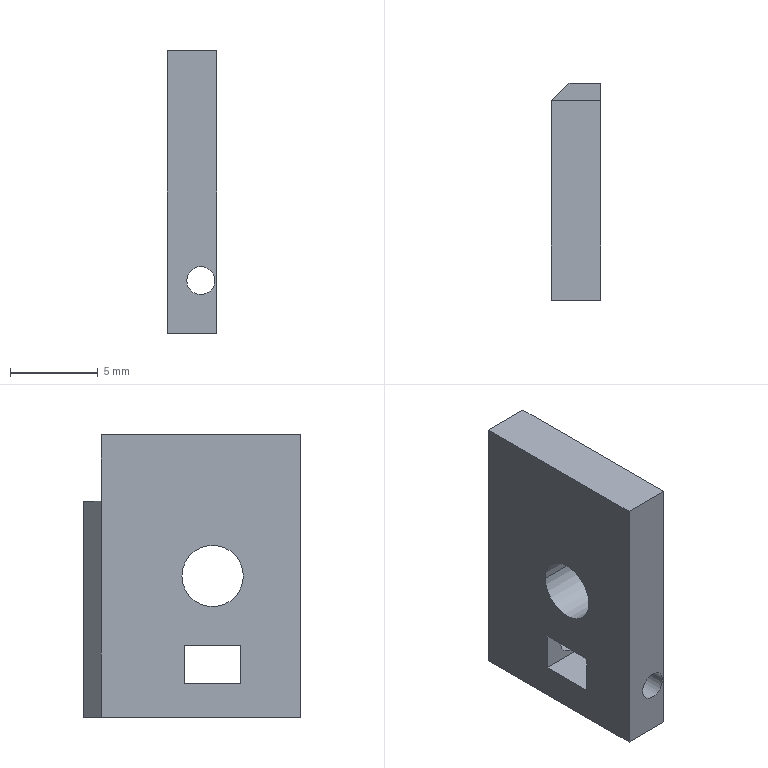Component | SolidWorks | 7.1.02.0001.00.00-0083-1 | 1 solid | 19 faces | box 2.8 x 12.35 x 16.1 mm | volume 475 mm3 | plane 13 | cylinder 6 | commonest cylinder face diameters 1.6 x4 3.5 x2
build123d program:
from build123d import *

# Parameters (mm, degrees)
SKETCH1_W           = 12.35
SKETCH1_H           = 16.1
SKETCH1_R           = 1.75
BOSS_EXTRUDE1_DEPTH = 2.8
SKETCH2_W           = 1
SKETCH2_H           = 3.8
CUT_EXTRUDE1_DEPTH  = 11.525
CHAMFER1_SIZE       = 1
SKETCH3_R           = 0.8
CUT_EXTRUDE2_DEPTH  = 16.005
SKETCH4_W           = 3.2
SKETCH4_H           = 2.2
CUT_EXTRUDE3_DEPTH  = 11.525


with BuildPart() as part:
    # Sketch1 → Boss-Extrude1 (new body)
    with BuildSketch(Plane.XY):
        Rectangle(SKETCH1_W, SKETCH1_H)
        with Locations((-1.175, 0)):
            Circle(SKETCH1_R, mode=Mode.SUBTRACT)
    extrude(amount=BOSS_EXTRUDE1_DEPTH)

    # Sketch2 → Cut-Extrude1 (cut, through all)
    with BuildSketch(Plane(origin=(0, 0, 0), x_dir=(-1, 0, 0), z_dir=(0, 0, -1))):
        with Locations((-5.675, 6.15)):
            Rectangle(SKETCH2_W, SKETCH2_H)
    extrude(amount=-CUT_EXTRUDE1_DEPTH, mode=Mode.SUBTRACT)

    # Chamfer1
    chamfer1_edges = [part.edges().sort_by_distance(p)[0] for p in [
        (6.175, -1.9, 0),
    ]]
    chamfer(chamfer1_edges, length=CHAMFER1_SIZE)

    # Sketch3 → Cut-Extrude2 (cut, through all)
    with BuildSketch(Plane.ZY.offset(6.175)):
        with Locations((1.9, -5.05)):
            Circle(SKETCH3_R)
    extrude(amount=-CUT_EXTRUDE2_DEPTH, mode=Mode.SUBTRACT)

    # Sketch4 → Cut-Extrude3 (cut, through all)
    with BuildSketch(Plane(origin=(0, 0, 0), x_dir=(-1, 0, 0), z_dir=(0, 0, -1))):
        with Locations((1.175, -5.05)):
            Rectangle(SKETCH4_W, SKETCH4_H)
    extrude(amount=-CUT_EXTRUDE3_DEPTH, mode=Mode.SUBTRACT)


solid = part.part

# Placed as in the assembly
solid = solid.moved(Location((-67.964, 9.491, 0), (90, 90, 0)))
STEP:
#1=COLOUR_RGB('',0.7922,0.8196,0.9333);
#2=FILL_AREA_STYLE_COLOUR('',#1);
#3=FILL_AREA_STYLE('',(#2));
#4=SURFACE_STYLE_FILL_AREA(#3);
#5=SURFACE_SIDE_STYLE('',(#4));
#6=SURFACE_STYLE_USAGE(.BOTH.,#5);
#7=PRESENTATION_STYLE_ASSIGNMENT((#6));
#8=CARTESIAN_POINT('',(-2.569,0.2644,-0.1988));
#9=VERTEX_POINT('',#8);
#10=CARTESIAN_POINT('',(-2.632,0.2644,-0.1988));
#11=VERTEX_POINT('',#10);
#12=CARTESIAN_POINT('',(-2.601,0.2644,-0.1988));
#13=DIRECTION('',(0.,1.,-0.));
#14=DIRECTION('',(0.,0.,-1.));
#15=AXIS2_PLACEMENT_3D('',#12,#13,#14);
#16=CIRCLE('',#15,0.0315);
#17=EDGE_CURVE('',#9,#11,#16,.T.);
#18=ORIENTED_EDGE('',*,*,#17,.T.);
#19=CARTESIAN_POINT('',(-2.632,0.1306,-0.1988));
#20=VERTEX_POINT('',#19);
#21=CARTESIAN_POINT('',(-2.632,0.6168,-0.1988));
#22=DIRECTION('',(-0.,-1.,-0.));
#23=VECTOR('',#22,39.37);
#24=LINE('',#21,#23);
#25=EDGE_CURVE('',#11,#20,#24,.T.);
#26=ORIENTED_EDGE('',*,*,#25,.T.);
#27=CARTESIAN_POINT('',(-2.569,0.1306,-0.1988));
#28=VERTEX_POINT('',#27);
#29=CARTESIAN_POINT('',(-2.601,0.1306,-0.1988));
#30=DIRECTION('',(-0.,-1.,-0.));
#31=DIRECTION('',(1.,0.,0.));
#32=AXIS2_PLACEMENT_3D('',#29,#30,#31);
#33=CIRCLE('',#32,0.0315);
#34=EDGE_CURVE('',#20,#28,#33,.T.);
#35=ORIENTED_EDGE('',*,*,#34,.T.);
#36=CARTESIAN_POINT('',(-2.569,0.6168,-0.1988));
#37=DIRECTION('',(-0.,-1.,-0.));
#38=VECTOR('',#37,39.37);
#39=LINE('',#36,#38);
#40=EDGE_CURVE('',#9,#28,#39,.T.);
#41=ORIENTED_EDGE('',*,*,#40,.F.);
#42=EDGE_LOOP('',(#18,#26,#35,#41));
#43=FACE_OUTER_BOUND('',#42,.T.);
#44=CARTESIAN_POINT('',(-2.601,0.6168,-0.1988));
#45=DIRECTION('',(-0.,-1.,-0.));
#46=DIRECTION('',(1.,0.,0.));
#47=AXIS2_PLACEMENT_3D('',#44,#45,#46);
#48=CYLINDRICAL_SURFACE('',#47,0.0315);
#49=ADVANCED_FACE('',(#43),#48,.F.);
#50=CARTESIAN_POINT('',(-2.566,0.2585,-0.));
#51=VERTEX_POINT('',#50);
#52=CARTESIAN_POINT('',(-2.566,0.3963,-0.));
#53=VERTEX_POINT('',#52);
#54=CARTESIAN_POINT('',(-2.566,0.3274,-0.));
#55=DIRECTION('',(1.,-0.,-0.));
#56=DIRECTION('',(0.,1.,0.));
#57=AXIS2_PLACEMENT_3D('',#54,#55,#56);
#58=CIRCLE('',#57,0.0689);
#59=EDGE_CURVE('',#51,#53,#58,.T.);
#60=ORIENTED_EDGE('',*,*,#59,.T.);
#61=CARTESIAN_POINT('',(-2.676,0.3963,-0.));
#62=VERTEX_POINT('',#61);
#63=CARTESIAN_POINT('',(-2.566,0.3963,-0.));
#64=DIRECTION('',(-1.,0.,0.));
#65=VECTOR('',#64,39.37);
#66=LINE('',#63,#65);
#67=EDGE_CURVE('',#53,#62,#66,.T.);
#68=ORIENTED_EDGE('',*,*,#67,.T.);
#69=CARTESIAN_POINT('',(-2.676,0.2585,-0.));
#70=VERTEX_POINT('',#69);
#71=CARTESIAN_POINT('',(-2.676,0.3274,-0.));
#72=DIRECTION('',(1.,-0.,-0.));
#73=DIRECTION('',(0.,1.,0.));
#74=AXIS2_PLACEMENT_3D('',#71,#72,#73);
#75=CIRCLE('',#74,0.0689);
#76=EDGE_CURVE('',#70,#62,#75,.T.);
#77=ORIENTED_EDGE('',*,*,#76,.F.);
#78=CARTESIAN_POINT('',(-2.566,0.2585,-0.));
#79=DIRECTION('',(-1.,0.,0.));
#80=VECTOR('',#79,39.37);
#81=LINE('',#78,#80);
#82=EDGE_CURVE('',#51,#70,#81,.T.);
#83=ORIENTED_EDGE('',*,*,#82,.F.);
#84=EDGE_LOOP('',(#60,#68,#77,#83));
#85=FACE_OUTER_BOUND('',#84,.T.);
#86=CARTESIAN_POINT('',(-2.566,0.3274,-0.));
#87=DIRECTION('',(-1.,0.,0.));
#88=DIRECTION('',(0.,-1.,-0.));
#89=AXIS2_PLACEMENT_3D('',#86,#87,#88);
#90=CYLINDRICAL_SURFACE('',#89,0.0689);
#91=ADVANCED_FACE('',(#85),#90,.F.);
#92=CARTESIAN_POINT('',(-2.632,0.6168,-0.1988));
#93=VERTEX_POINT('',#92);
#94=CARTESIAN_POINT('',(-2.569,0.6168,-0.1988));
#95=VERTEX_POINT('',#94);
#96=CARTESIAN_POINT('',(-2.601,0.6168,-0.1988));
#97=DIRECTION('',(-0.,-1.,-0.));
#98=DIRECTION('',(1.,0.,0.));
#99=AXIS2_PLACEMENT_3D('',#96,#97,#98);
#100=CIRCLE('',#99,0.0315);
#101=EDGE_CURVE('',#93,#95,#100,.T.);
#102=ORIENTED_EDGE('',*,*,#101,.F.);
#103=CARTESIAN_POINT('',(-2.632,0.3904,-0.1988));
#104=VERTEX_POINT('',#103);
#105=CARTESIAN_POINT('',(-2.632,0.6168,-0.1988));
#106=DIRECTION('',(-0.,-1.,-0.));
#107=VECTOR('',#106,39.37);
#108=LINE('',#105,#107);
#109=EDGE_CURVE('',#93,#104,#108,.T.);
#110=ORIENTED_EDGE('',*,*,#109,.T.);
#111=CARTESIAN_POINT('',(-2.569,0.3904,-0.1988));
#112=VERTEX_POINT('',#111);
#113=CARTESIAN_POINT('',(-2.601,0.3904,-0.1988));
#114=DIRECTION('',(-0.,-1.,-0.));
#115=DIRECTION('',(-1.,0.,0.));
#116=AXIS2_PLACEMENT_3D('',#113,#114,#115);
#117=CIRCLE('',#116,0.0315);
#118=EDGE_CURVE('',#104,#112,#117,.T.);
#119=ORIENTED_EDGE('',*,*,#118,.T.);
#120=CARTESIAN_POINT('',(-2.569,0.6168,-0.1988));
#121=DIRECTION('',(-0.,-1.,-0.));
#122=VECTOR('',#121,39.37);
#123=LINE('',#120,#122);
#124=EDGE_CURVE('',#95,#112,#123,.T.);
#125=ORIENTED_EDGE('',*,*,#124,.F.);
#126=EDGE_LOOP('',(#102,#110,#119,#125));
#127=FACE_OUTER_BOUND('',#126,.T.);
#128=CARTESIAN_POINT('',(-2.601,0.6168,-0.1988));
#129=DIRECTION('',(-0.,-1.,-0.));
#130=DIRECTION('',(1.,0.,0.));
#131=AXIS2_PLACEMENT_3D('',#128,#129,#130);
#132=CYLINDRICAL_SURFACE('',#131,0.0315);
#133=ADVANCED_FACE('',(#127),#132,.F.);
#134=ORIENTED_EDGE('',*,*,#109,.F.);
#135=CARTESIAN_POINT('',(-2.601,0.6168,-0.1988));
#136=DIRECTION('',(-0.,-1.,-0.));
#137=DIRECTION('',(1.,0.,0.));
#138=AXIS2_PLACEMENT_3D('',#135,#136,#137);
#139=CIRCLE('',#138,0.0315);
#140=EDGE_CURVE('',#95,#93,#139,.T.);
#141=ORIENTED_EDGE('',*,*,#140,.F.);
#142=ORIENTED_EDGE('',*,*,#124,.T.);
#143=CARTESIAN_POINT('',(-2.601,0.3904,-0.1988));
#144=DIRECTION('',(-0.,-1.,-0.));
#145=DIRECTION('',(-1.,0.,0.));
#146=AXIS2_PLACEMENT_3D('',#143,#144,#145);
#147=CIRCLE('',#146,0.0315);
#148=EDGE_CURVE('',#112,#104,#147,.T.);
#149=ORIENTED_EDGE('',*,*,#148,.T.);
#150=EDGE_LOOP('',(#134,#141,#142,#149));
#151=FACE_OUTER_BOUND('',#150,.T.);
#152=CARTESIAN_POINT('',(-2.601,0.6168,-0.1988));
#153=DIRECTION('',(-0.,-1.,-0.));
#154=DIRECTION('',(1.,0.,0.));
#155=AXIS2_PLACEMENT_3D('',#152,#153,#154);
#156=CYLINDRICAL_SURFACE('',#155,0.0315);
#157=ADVANCED_FACE('',(#151),#156,.F.);
#158=CARTESIAN_POINT('',(-2.566,0.3904,-0.1555));
#159=VERTEX_POINT('',#158);
#160=CARTESIAN_POINT('',(-2.566,0.3904,-0.2421));
#161=VERTEX_POINT('',#160);
#162=CARTESIAN_POINT('',(-2.566,0.3904,-0.1555));
#163=DIRECTION('',(-0.,0.,-1.));
#164=VECTOR('',#163,39.37);
#165=LINE('',#162,#164);
#166=EDGE_CURVE('',#159,#161,#165,.T.);
#167=ORIENTED_EDGE('',*,*,#166,.T.);
#168=CARTESIAN_POINT('',(-2.566,0.2644,-0.2421));
#169=VERTEX_POINT('',#168);
#170=CARTESIAN_POINT('',(-2.566,0.3904,-0.2421));
#171=DIRECTION('',(-0.,-1.,-0.));
#172=VECTOR('',#171,39.37);
#173=LINE('',#170,#172);
#174=EDGE_CURVE('',#161,#169,#173,.T.);
#175=ORIENTED_EDGE('',*,*,#174,.T.);
#176=CARTESIAN_POINT('',(-2.566,0.2644,-0.1555));
#177=VERTEX_POINT('',#176);
#178=CARTESIAN_POINT('',(-2.566,0.2644,-0.1555));
#179=DIRECTION('',(0.,0.,1.));
#180=VECTOR('',#179,39.37);
#181=LINE('',#178,#180);
#182=EDGE_CURVE('',#169,#177,#181,.T.);
#183=ORIENTED_EDGE('',*,*,#182,.T.);
#184=CARTESIAN_POINT('',(-2.566,0.3904,-0.1555));
#185=DIRECTION('',(0.,1.,0.));
#186=VECTOR('',#185,39.37);
#187=LINE('',#184,#186);
#188=EDGE_CURVE('',#177,#159,#187,.T.);
#189=ORIENTED_EDGE('',*,*,#188,.T.);
#190=EDGE_LOOP('',(#167,#175,#183,#189));
#191=FACE_BOUND('',#190,.T.);
#192=CARTESIAN_POINT('',(-2.566,0.5774,0.1673));
#193=VERTEX_POINT('',#192);
#194=CARTESIAN_POINT('',(-2.566,0.5774,0.3169));
#195=VERTEX_POINT('',#194);
#196=CARTESIAN_POINT('',(-2.566,0.5774,0.1673));
#197=DIRECTION('',(0.,-0.,1.));
#198=VECTOR('',#197,39.37);
#199=LINE('',#196,#198);
#200=EDGE_CURVE('',#193,#195,#199,.T.);
#201=ORIENTED_EDGE('',*,*,#200,.T.);
#202=CARTESIAN_POINT('',(-2.566,0.1306,0.3169));
#203=VERTEX_POINT('',#202);
#204=CARTESIAN_POINT('',(-2.566,0.1306,0.3169));
#205=DIRECTION('',(-0.,-1.,-0.));
#206=VECTOR('',#205,39.37);
#207=LINE('',#204,#206);
#208=EDGE_CURVE('',#195,#203,#207,.T.);
#209=ORIENTED_EDGE('',*,*,#208,.T.);
#210=CARTESIAN_POINT('',(-2.566,0.1306,-0.3169));
#211=VERTEX_POINT('',#210);
#212=CARTESIAN_POINT('',(-2.566,0.1306,0.3169));
#213=DIRECTION('',(-0.,0.,-1.));
#214=VECTOR('',#213,39.37);
#215=LINE('',#212,#214);
#216=EDGE_CURVE('',#203,#211,#215,.T.);
#217=ORIENTED_EDGE('',*,*,#216,.T.);
#218=CARTESIAN_POINT('',(-2.566,0.6168,-0.3169));
#219=VERTEX_POINT('',#218);
#220=CARTESIAN_POINT('',(-2.566,0.1306,-0.3169));
#221=DIRECTION('',(0.,1.,0.));
#222=VECTOR('',#221,39.37);
#223=LINE('',#220,#222);
#224=EDGE_CURVE('',#211,#219,#223,.T.);
#225=ORIENTED_EDGE('',*,*,#224,.T.);
#226=CARTESIAN_POINT('',(-2.566,0.6168,0.1673));
#227=VERTEX_POINT('',#226);
#228=CARTESIAN_POINT('',(-2.566,0.6168,0.3169));
#229=DIRECTION('',(0.,-0.,1.));
#230=VECTOR('',#229,39.37);
#231=LINE('',#228,#230);
#232=EDGE_CURVE('',#219,#227,#231,.T.);
#233=ORIENTED_EDGE('',*,*,#232,.T.);
#234=CARTESIAN_POINT('',(-2.566,0.6168,0.1673));
#235=DIRECTION('',(-0.,-1.,-0.));
#236=VECTOR('',#235,39.37);
#237=LINE('',#234,#236);
#238=EDGE_CURVE('',#227,#193,#237,.T.);
#239=ORIENTED_EDGE('',*,*,#238,.T.);
#240=EDGE_LOOP('',(#201,#209,#217,#225,#233,#239));
#241=FACE_OUTER_BOUND('',#240,.T.);
#242=ORIENTED_EDGE('',*,*,#59,.F.);
#243=CARTESIAN_POINT('',(-2.566,0.3274,-0.));
#244=DIRECTION('',(1.,-0.,-0.));
#245=DIRECTION('',(0.,1.,0.));
#246=AXIS2_PLACEMENT_3D('',#243,#244,#245);
#247=CIRCLE('',#246,0.0689);
#248=EDGE_CURVE('',#53,#51,#247,.T.);
#249=ORIENTED_EDGE('',*,*,#248,.F.);
#250=EDGE_LOOP('',(#242,#249));
#251=FACE_BOUND('',#250,.T.);
#252=CARTESIAN_POINT('',(-2.566,0.3737,-0.));
#253=DIRECTION('',(1.,-0.,-0.));
#254=DIRECTION('',(0.,1.,0.));
#255=AXIS2_PLACEMENT_3D('',#252,#253,#254);
#256=PLANE('',#255);
#257=ADVANCED_FACE('',(#191,#241,#251),#256,.T.);
#258=CARTESIAN_POINT('',(-2.676,0.3904,-0.2421));
#259=VERTEX_POINT('',#258);
#260=CARTESIAN_POINT('',(-2.676,0.2644,-0.2421));
#261=VERTEX_POINT('',#260);
#262=CARTESIAN_POINT('',(-2.676,0.3904,-0.2421));
#263=DIRECTION('',(-0.,-1.,-0.));
#264=VECTOR('',#263,39.37);
#265=LINE('',#262,#264);
#266=EDGE_CURVE('',#259,#261,#265,.T.);
#267=ORIENTED_EDGE('',*,*,#266,.F.);
#268=CARTESIAN_POINT('',(-2.676,0.3904,-0.1555));
#269=VERTEX_POINT('',#268);
#270=CARTESIAN_POINT('',(-2.676,0.3904,-0.1555));
#271=DIRECTION('',(-0.,0.,-1.));
#272=VECTOR('',#271,39.37);
#273=LINE('',#270,#272);
#274=EDGE_CURVE('',#269,#259,#273,.T.);
#275=ORIENTED_EDGE('',*,*,#274,.F.);
#276=CARTESIAN_POINT('',(-2.676,0.2644,-0.1555));
#277=VERTEX_POINT('',#276);
#278=CARTESIAN_POINT('',(-2.676,0.3904,-0.1555));
#279=DIRECTION('',(0.,1.,0.));
#280=VECTOR('',#279,39.37);
#281=LINE('',#278,#280);
#282=EDGE_CURVE('',#277,#269,#281,.T.);
#283=ORIENTED_EDGE('',*,*,#282,.F.);
#284=CARTESIAN_POINT('',(-2.676,0.2644,-0.1555));
#285=DIRECTION('',(0.,0.,1.));
#286=VECTOR('',#285,39.37);
#287=LINE('',#284,#286);
#288=EDGE_CURVE('',#261,#277,#287,.T.);
#289=ORIENTED_EDGE('',*,*,#288,.F.);
#290=EDGE_LOOP('',(#267,#275,#283,#289));
#291=FACE_BOUND('',#290,.T.);
#292=CARTESIAN_POINT('',(-2.676,0.5774,0.1673));
#293=VERTEX_POINT('',#292);
#294=CARTESIAN_POINT('',(-2.676,0.5774,0.3169));
#295=VERTEX_POINT('',#294);
#296=CARTESIAN_POINT('',(-2.676,0.5774,0.1673));
#297=DIRECTION('',(0.,-0.,1.));
#298=VECTOR('',#297,39.37);
#299=LINE('',#296,#298);
#300=EDGE_CURVE('',#293,#295,#299,.T.);
#301=ORIENTED_EDGE('',*,*,#300,.F.);
#302=CARTESIAN_POINT('',(-2.676,0.5774,-0.3169));
#303=VERTEX_POINT('',#302);
#304=CARTESIAN_POINT('',(-2.676,0.5774,-0.));
#305=DIRECTION('',(-0.,0.,-1.));
#306=VECTOR('',#305,39.37);
#307=LINE('',#304,#306);
#308=EDGE_CURVE('',#293,#303,#307,.T.);
#309=ORIENTED_EDGE('',*,*,#308,.T.);
#310=CARTESIAN_POINT('',(-2.676,0.1306,-0.3169));
#311=VERTEX_POINT('',#310);
#312=CARTESIAN_POINT('',(-2.676,0.1306,-0.3169));
#313=DIRECTION('',(0.,1.,0.));
#314=VECTOR('',#313,39.37);
#315=LINE('',#312,#314);
#316=EDGE_CURVE('',#311,#303,#315,.T.);
#317=ORIENTED_EDGE('',*,*,#316,.F.);
#318=CARTESIAN_POINT('',(-2.676,0.1306,0.3169));
#319=VERTEX_POINT('',#318);
#320=CARTESIAN_POINT('',(-2.676,0.1306,0.3169));
#321=DIRECTION('',(-0.,0.,-1.));
#322=VECTOR('',#321,39.37);
#323=LINE('',#320,#322);
#324=EDGE_CURVE('',#319,#311,#323,.T.);
#325=ORIENTED_EDGE('',*,*,#324,.F.);
#326=CARTESIAN_POINT('',(-2.676,0.1306,0.3169));
#327=DIRECTION('',(-0.,-1.,-0.));
#328=VECTOR('',#327,39.37);
#329=LINE('',#326,#328);
#330=EDGE_CURVE('',#295,#319,#329,.T.);
#331=ORIENTED_EDGE('',*,*,#330,.F.);
#332=EDGE_LOOP('',(#301,#309,#317,#325,#331));
#333=FACE_OUTER_BOUND('',#332,.T.);
#334=ORIENTED_EDGE('',*,*,#76,.T.);
#335=CARTESIAN_POINT('',(-2.676,0.3274,-0.));
#336=DIRECTION('',(1.,-0.,-0.));
#337=DIRECTION('',(0.,1.,0.));
#338=AXIS2_PLACEMENT_3D('',#335,#336,#337);
#339=CIRCLE('',#338,0.0689);
#340=EDGE_CURVE('',#62,#70,#339,.T.);
#341=ORIENTED_EDGE('',*,*,#340,.T.);
#342=EDGE_LOOP('',(#334,#341));
#343=FACE_BOUND('',#342,.T.);
#344=CARTESIAN_POINT('',(-2.676,0.3737,-0.));
#345=DIRECTION('',(1.,-0.,-0.));
#346=DIRECTION('',(0.,1.,0.));
#347=AXIS2_PLACEMENT_3D('',#344,#345,#346);
#348=PLANE('',#347);
#349=ADVANCED_FACE('',(#291,#333,#343),#348,.F.);
#350=CARTESIAN_POINT('',(-2.601,0.1306,-0.1988));
#351=DIRECTION('',(-0.,-1.,-0.));
#352=DIRECTION('',(1.,0.,0.));
#353=AXIS2_PLACEMENT_3D('',#350,#351,#352);
#354=CIRCLE('',#353,0.0315);
#355=EDGE_CURVE('',#28,#20,#354,.T.);
#356=ORIENTED_EDGE('',*,*,#355,.F.);
#357=ORIENTED_EDGE('',*,*,#34,.F.);
#358=EDGE_LOOP('',(#356,#357));
#359=FACE_BOUND('',#358,.T.);
#360=ORIENTED_EDGE('',*,*,#324,.T.);
#361=CARTESIAN_POINT('',(-2.566,0.1306,-0.3169));
#362=DIRECTION('',(-1.,0.,0.));
#363=VECTOR('',#362,39.37);
#364=LINE('',#361,#363);
#365=EDGE_CURVE('',#211,#311,#364,.T.);
#366=ORIENTED_EDGE('',*,*,#365,.F.);
#367=ORIENTED_EDGE('',*,*,#216,.F.);
#368=CARTESIAN_POINT('',(-2.566,0.1306,0.3169));
#369=DIRECTION('',(-1.,0.,0.));
#370=VECTOR('',#369,39.37);
#371=LINE('',#368,#370);
#372=EDGE_CURVE('',#203,#319,#371,.T.);
#373=ORIENTED_EDGE('',*,*,#372,.T.);
#374=EDGE_LOOP('',(#360,#366,#367,#373));
#375=FACE_OUTER_BOUND('',#374,.T.);
#376=CARTESIAN_POINT('',(-2.566,0.1306,0.3169));
#377=DIRECTION('',(0.,1.,0.));
#378=DIRECTION('',(-1.,0.,0.));
#379=AXIS2_PLACEMENT_3D('',#376,#377,#378);
#380=PLANE('',#379);
#381=ADVANCED_FACE('',(#359,#375),#380,.F.);
#382=ORIENTED_EDGE('',*,*,#316,.T.);
#383=CARTESIAN_POINT('',(-2.636,0.6168,-0.3169));
#384=VERTEX_POINT('',#383);
#385=CARTESIAN_POINT('',(-2.636,0.6168,-0.3169));
#386=DIRECTION('',(0.7071,0.7071,0.));
#387=VECTOR('',#386,39.37);
#388=LINE('',#385,#387);
#389=EDGE_CURVE('',#303,#384,#388,.T.);
#390=ORIENTED_EDGE('',*,*,#389,.T.);
#391=CARTESIAN_POINT('',(-2.566,0.6168,-0.3169));
#392=DIRECTION('',(-1.,0.,0.));
#393=VECTOR('',#392,39.37);
#394=LINE('',#391,#393);
#395=EDGE_CURVE('',#219,#384,#394,.T.);
#396=ORIENTED_EDGE('',*,*,#395,.F.);
#397=ORIENTED_EDGE('',*,*,#224,.F.);
#398=ORIENTED_EDGE('',*,*,#365,.T.);
#399=EDGE_LOOP('',(#382,#390,#396,#397,#398));
#400=FACE_OUTER_BOUND('',#399,.T.);
#401=CARTESIAN_POINT('',(-2.566,0.1306,-0.3169));
#402=DIRECTION('',(0.,-0.,1.));
#403=DIRECTION('',(1.,-0.,-0.));
#404=AXIS2_PLACEMENT_3D('',#401,#402,#403);
#405=PLANE('',#404);
#406=ADVANCED_FACE('',(#400),#405,.F.);
#407=ORIENTED_EDGE('',*,*,#140,.T.);
#408=ORIENTED_EDGE('',*,*,#101,.T.);
#409=EDGE_LOOP('',(#407,#408));
#410=FACE_BOUND('',#409,.T.);
#411=ORIENTED_EDGE('',*,*,#395,.T.);
#412=CARTESIAN_POINT('',(-2.636,0.6168,0.1673));
#413=VERTEX_POINT('',#412);
#414=CARTESIAN_POINT('',(-2.636,0.6168,0.3169));
#415=DIRECTION('',(0.,-0.,1.));
#416=VECTOR('',#415,39.37);
#417=LINE('',#414,#416);
#418=EDGE_CURVE('',#384,#413,#417,.T.);
#419=ORIENTED_EDGE('',*,*,#418,.T.);
#420=CARTESIAN_POINT('',(-2.566,0.6168,0.1673));
#421=DIRECTION('',(-1.,0.,0.));
#422=VECTOR('',#421,39.37);
#423=LINE('',#420,#422);
#424=EDGE_CURVE('',#227,#413,#423,.T.);
#425=ORIENTED_EDGE('',*,*,#424,.F.);
#426=ORIENTED_EDGE('',*,*,#232,.F.);
#427=EDGE_LOOP('',(#411,#419,#425,#426));
#428=FACE_OUTER_BOUND('',#427,.T.);
#429=CARTESIAN_POINT('',(-2.566,0.6168,0.3169));
#430=DIRECTION('',(-0.,-1.,-0.));
#431=DIRECTION('',(1.,-0.,-0.));
#432=AXIS2_PLACEMENT_3D('',#429,#430,#431);
#433=PLANE('',#432);
#434=ADVANCED_FACE('',(#410,#428),#433,.F.);
#435=ORIENTED_EDGE('',*,*,#208,.F.);
#436=CARTESIAN_POINT('',(-2.566,0.5774,0.3169));
#437=DIRECTION('',(-1.,0.,0.));
#438=VECTOR('',#437,39.37);
#439=LINE('',#436,#438);
#440=EDGE_CURVE('',#195,#295,#439,.T.);
#441=ORIENTED_EDGE('',*,*,#440,.T.);
#442=ORIENTED_EDGE('',*,*,#330,.T.);
#443=ORIENTED_EDGE('',*,*,#372,.F.);
#444=EDGE_LOOP('',(#435,#441,#442,#443));
#445=FACE_OUTER_BOUND('',#444,.T.);
#446=CARTESIAN_POINT('',(-2.566,0.1306,0.3169));
#447=DIRECTION('',(-0.,0.,-1.));
#448=DIRECTION('',(-1.,0.,0.));
#449=AXIS2_PLACEMENT_3D('',#446,#447,#448);
#450=PLANE('',#449);
#451=ADVANCED_FACE('',(#445),#450,.F.);
#452=ORIENTED_EDGE('',*,*,#67,.F.);
#453=ORIENTED_EDGE('',*,*,#248,.T.);
#454=ORIENTED_EDGE('',*,*,#82,.T.);
#455=ORIENTED_EDGE('',*,*,#340,.F.);
#456=EDGE_LOOP('',(#452,#453,#454,#455));
#457=FACE_OUTER_BOUND('',#456,.T.);
#458=CARTESIAN_POINT('',(-2.566,0.3274,-0.));
#459=DIRECTION('',(-1.,0.,0.));
#460=DIRECTION('',(0.,-1.,-0.));
#461=AXIS2_PLACEMENT_3D('',#458,#459,#460);
#462=CYLINDRICAL_SURFACE('',#461,0.0689);
#463=ADVANCED_FACE('',(#457),#462,.F.);
#464=ORIENTED_EDGE('',*,*,#300,.T.);
#465=ORIENTED_EDGE('',*,*,#440,.F.);
#466=ORIENTED_EDGE('',*,*,#200,.F.);
#467=CARTESIAN_POINT('',(-2.566,0.5774,0.1673));
#468=DIRECTION('',(-1.,0.,0.));
#469=VECTOR('',#468,39.37);
#470=LINE('',#467,#469);
#471=EDGE_CURVE('',#193,#293,#470,.T.);
#472=ORIENTED_EDGE('',*,*,#471,.T.);
#473=EDGE_LOOP('',(#464,#465,#466,#472));
#474=FACE_OUTER_BOUND('',#473,.T.);
#475=CARTESIAN_POINT('',(-2.566,0.5774,0.1673));
#476=DIRECTION('',(-0.,-1.,-0.));
#477=DIRECTION('',(1.,-0.,-0.));
#478=AXIS2_PLACEMENT_3D('',#475,#476,#477);
#479=PLANE('',#478);
#480=ADVANCED_FACE('',(#474),#479,.F.);
#481=ORIENTED_EDGE('',*,*,#424,.T.);
#482=CARTESIAN_POINT('',(-2.636,0.6168,0.1673));
#483=DIRECTION('',(-0.7071,-0.7071,-0.));
#484=VECTOR('',#483,39.37);
#485=LINE('',#482,#484);
#486=EDGE_CURVE('',#413,#293,#485,.T.);
#487=ORIENTED_EDGE('',*,*,#486,.T.);
#488=ORIENTED_EDGE('',*,*,#471,.F.);
#489=ORIENTED_EDGE('',*,*,#238,.F.);
#490=EDGE_LOOP('',(#481,#487,#488,#489));
#491=FACE_OUTER_BOUND('',#490,.T.);
#492=CARTESIAN_POINT('',(-2.566,0.6168,0.1673));
#493=DIRECTION('',(-0.,0.,-1.));
#494=DIRECTION('',(-1.,0.,0.));
#495=AXIS2_PLACEMENT_3D('',#492,#493,#494);
#496=PLANE('',#495);
#497=ADVANCED_FACE('',(#491),#496,.F.);
#498=ORIENTED_EDGE('',*,*,#389,.F.);
#499=ORIENTED_EDGE('',*,*,#308,.F.);
#500=ORIENTED_EDGE('',*,*,#486,.F.);
#501=ORIENTED_EDGE('',*,*,#418,.F.);
#502=EDGE_LOOP('',(#498,#499,#500,#501));
#503=FACE_OUTER_BOUND('',#502,.T.);
#504=CARTESIAN_POINT('',(-2.636,0.6168,0.3169));
#505=DIRECTION('',(0.7071,-0.7071,-0.));
#506=DIRECTION('',(0.,-0.,1.));
#507=AXIS2_PLACEMENT_3D('',#504,#505,#506);
#508=PLANE('',#507);
#509=ADVANCED_FACE('',(#503),#508,.F.);
#510=ORIENTED_EDGE('',*,*,#25,.F.);
#511=CARTESIAN_POINT('',(-2.601,0.2644,-0.1988));
#512=DIRECTION('',(0.,1.,-0.));
#513=DIRECTION('',(0.,0.,-1.));
#514=AXIS2_PLACEMENT_3D('',#511,#512,#513);
#515=CIRCLE('',#514,0.0315);
#516=EDGE_CURVE('',#11,#9,#515,.T.);
#517=ORIENTED_EDGE('',*,*,#516,.T.);
#518=ORIENTED_EDGE('',*,*,#40,.T.);
#519=ORIENTED_EDGE('',*,*,#355,.T.);
#520=EDGE_LOOP('',(#510,#517,#518,#519));
#521=FACE_OUTER_BOUND('',#520,.T.);
#522=CARTESIAN_POINT('',(-2.601,0.6168,-0.1988));
#523=DIRECTION('',(-0.,-1.,-0.));
#524=DIRECTION('',(1.,0.,0.));
#525=AXIS2_PLACEMENT_3D('',#522,#523,#524);
#526=CYLINDRICAL_SURFACE('',#525,0.0315);
#527=ADVANCED_FACE('',(#521),#526,.F.);
#528=ORIENTED_EDGE('',*,*,#274,.T.);
#529=CARTESIAN_POINT('',(-2.566,0.3904,-0.2421));
#530=DIRECTION('',(-1.,0.,0.));
#531=VECTOR('',#530,39.37);
#532=LINE('',#529,#531);
#533=EDGE_CURVE('',#161,#259,#532,.T.);
#534=ORIENTED_EDGE('',*,*,#533,.F.);
#535=ORIENTED_EDGE('',*,*,#166,.F.);
#536=CARTESIAN_POINT('',(-2.566,0.3904,-0.1555));
#537=DIRECTION('',(-1.,0.,0.));
#538=VECTOR('',#537,39.37);
#539=LINE('',#536,#538);
#540=EDGE_CURVE('',#159,#269,#539,.T.);
#541=ORIENTED_EDGE('',*,*,#540,.T.);
#542=EDGE_LOOP('',(#528,#534,#535,#541));
#543=FACE_OUTER_BOUND('',#542,.T.);
#544=ORIENTED_EDGE('',*,*,#148,.F.);
#545=ORIENTED_EDGE('',*,*,#118,.F.);
#546=EDGE_LOOP('',(#544,#545));
#547=FACE_BOUND('',#546,.T.);
#548=CARTESIAN_POINT('',(-2.566,0.3904,-0.1555));
#549=DIRECTION('',(0.,1.,0.));
#550=DIRECTION('',(-1.,0.,0.));
#551=AXIS2_PLACEMENT_3D('',#548,#549,#550);
#552=PLANE('',#551);
#553=ADVANCED_FACE('',(#543,#547),#552,.F.);
#554=ORIENTED_EDGE('',*,*,#288,.T.);
#555=CARTESIAN_POINT('',(-2.566,0.2644,-0.1555));
#556=DIRECTION('',(-1.,0.,0.));
#557=VECTOR('',#556,39.37);
#558=LINE('',#555,#557);
#559=EDGE_CURVE('',#177,#277,#558,.T.);
#560=ORIENTED_EDGE('',*,*,#559,.F.);
#561=ORIENTED_EDGE('',*,*,#182,.F.);
#562=CARTESIAN_POINT('',(-2.566,0.2644,-0.2421));
#563=DIRECTION('',(-1.,0.,0.));
#564=VECTOR('',#563,39.37);
#565=LINE('',#562,#564);
#566=EDGE_CURVE('',#169,#261,#565,.T.);
#567=ORIENTED_EDGE('',*,*,#566,.T.);
#568=EDGE_LOOP('',(#554,#560,#561,#567));
#569=FACE_OUTER_BOUND('',#568,.T.);
#570=ORIENTED_EDGE('',*,*,#17,.F.);
#571=ORIENTED_EDGE('',*,*,#516,.F.);
#572=EDGE_LOOP('',(#570,#571));
#573=FACE_BOUND('',#572,.T.);
#574=CARTESIAN_POINT('',(-2.566,0.2644,-0.1555));
#575=DIRECTION('',(-0.,-1.,0.));
#576=DIRECTION('',(-0.,-0.,-1.));
#577=AXIS2_PLACEMENT_3D('',#574,#575,#576);
#578=PLANE('',#577);
#579=ADVANCED_FACE('',(#569,#573),#578,.F.);
#580=ORIENTED_EDGE('',*,*,#282,.T.);
#581=ORIENTED_EDGE('',*,*,#540,.F.);
#582=ORIENTED_EDGE('',*,*,#188,.F.);
#583=ORIENTED_EDGE('',*,*,#559,.T.);
#584=EDGE_LOOP('',(#580,#581,#582,#583));
#585=FACE_OUTER_BOUND('',#584,.T.);
#586=CARTESIAN_POINT('',(-2.566,0.3904,-0.1555));
#587=DIRECTION('',(0.,-0.,1.));
#588=DIRECTION('',(1.,-0.,-0.));
#589=AXIS2_PLACEMENT_3D('',#586,#587,#588);
#590=PLANE('',#589);
#591=ADVANCED_FACE('',(#585),#590,.F.);
#592=ORIENTED_EDGE('',*,*,#266,.T.);
#593=ORIENTED_EDGE('',*,*,#566,.F.);
#594=ORIENTED_EDGE('',*,*,#174,.F.);
#595=ORIENTED_EDGE('',*,*,#533,.T.);
#596=EDGE_LOOP('',(#592,#593,#594,#595));
#597=FACE_OUTER_BOUND('',#596,.T.);
#598=CARTESIAN_POINT('',(-2.566,0.3904,-0.2421));
#599=DIRECTION('',(-0.,0.,-1.));
#600=DIRECTION('',(-1.,0.,0.));
#601=AXIS2_PLACEMENT_3D('',#598,#599,#600);
#602=PLANE('',#601);
#603=ADVANCED_FACE('',(#597),#602,.F.);
#604=CLOSED_SHELL('',(#49,#91,#133,#157,#257,#349,#381,#406,#434,#451,#463,#480,#497,#509,#527,#553,#579,#591,#603));
#605=MANIFOLD_SOLID_BREP('',#604);
#606=STYLED_ITEM('',(#7),#605);
#607=PRESENTATION_LAYER_ASSIGNMENT('','',(#606));
#608=CARTESIAN_POINT('',(0.,0.,0.));
#609=DIRECTION('',(0.,0.,1.));
#610=DIRECTION('',(1.,0.,0.));
#611=AXIS2_PLACEMENT_3D('',#608,#609,#610);
#612=(LENGTH_UNIT()NAMED_UNIT(*)SI_UNIT($,.METRE.));
#613=LENGTH_MEASURE_WITH_UNIT(LENGTH_MEASURE(0.0254),#612);
#614=DIMENSIONAL_EXPONENTS(1.,0.,0.,0.,0.,0.,0.);
#615=(CONVERSION_BASED_UNIT('',#613)LENGTH_UNIT()NAMED_UNIT(#614));
#616=UNCERTAINTY_MEASURE_WITH_UNIT(LENGTH_MEASURE(0.00001),#615,'','');
#617=(NAMED_UNIT(*)PLANE_ANGLE_UNIT()SI_UNIT($,.RADIAN.));
#618=(NAMED_UNIT(*)SI_UNIT($,.STERADIAN.)SOLID_ANGLE_UNIT());
#619=(GEOMETRIC_REPRESENTATION_CONTEXT(3)GLOBAL_UNCERTAINTY_ASSIGNED_CONTEXT((#616))GLOBAL_UNIT_ASSIGNED_CONTEXT((#615,#617,#618))REPRESENTATION_CONTEXT('',''));
#620=ADVANCED_BREP_SHAPE_REPRESENTATION('',(#605,#611),#619);
#621=(LENGTH_UNIT()NAMED_UNIT(*)SI_UNIT($,.METRE.));
#622=LENGTH_MEASURE_WITH_UNIT(LENGTH_MEASURE(0.0254),#621);
#623=DIMENSIONAL_EXPONENTS(1.,0.,0.,0.,0.,0.,0.);
#624=(CONVERSION_BASED_UNIT('',#622)LENGTH_UNIT()NAMED_UNIT(#623));
#625=UNCERTAINTY_MEASURE_WITH_UNIT(LENGTH_MEASURE(0.00001),#624,'','');
#626=(NAMED_UNIT(*)PLANE_ANGLE_UNIT()SI_UNIT($,.RADIAN.));
#627=(NAMED_UNIT(*)SI_UNIT($,.STERADIAN.)SOLID_ANGLE_UNIT());
#628=(GEOMETRIC_REPRESENTATION_CONTEXT(3)GLOBAL_UNCERTAINTY_ASSIGNED_CONTEXT((#625))GLOBAL_UNIT_ASSIGNED_CONTEXT((#624,#626,#627))REPRESENTATION_CONTEXT('',''));
#629=MECHANICAL_DESIGN_GEOMETRIC_PRESENTATION_REPRESENTATION('',(#606),#628);